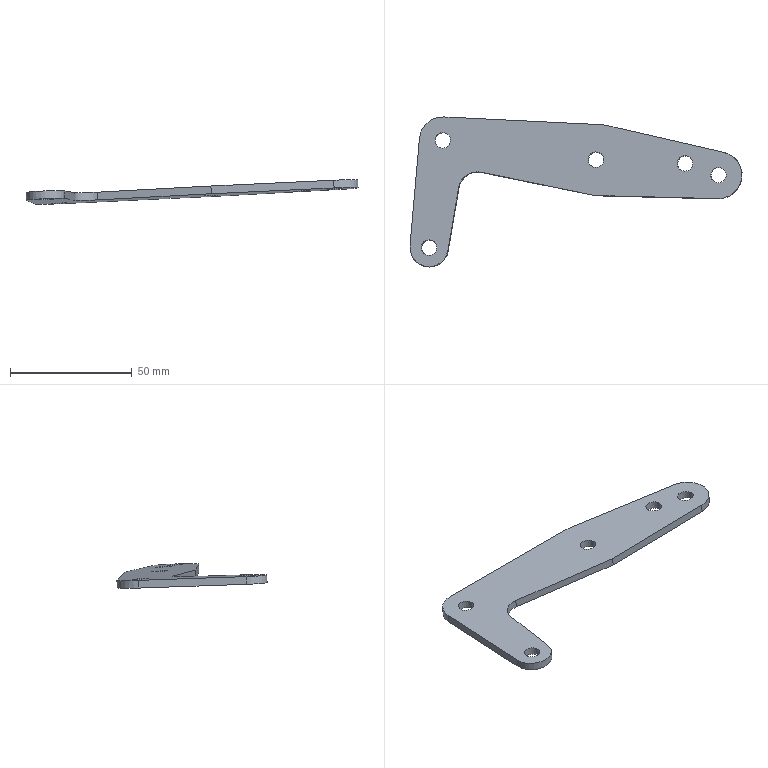Component | NX | RIOSTRA_A | 1 solid | 17 faces | volume 11559 mm3 | cylinder 9 | plane 8 | commonest cylinder face diameters 6.35 x5 15.748 x2 19.304 x2